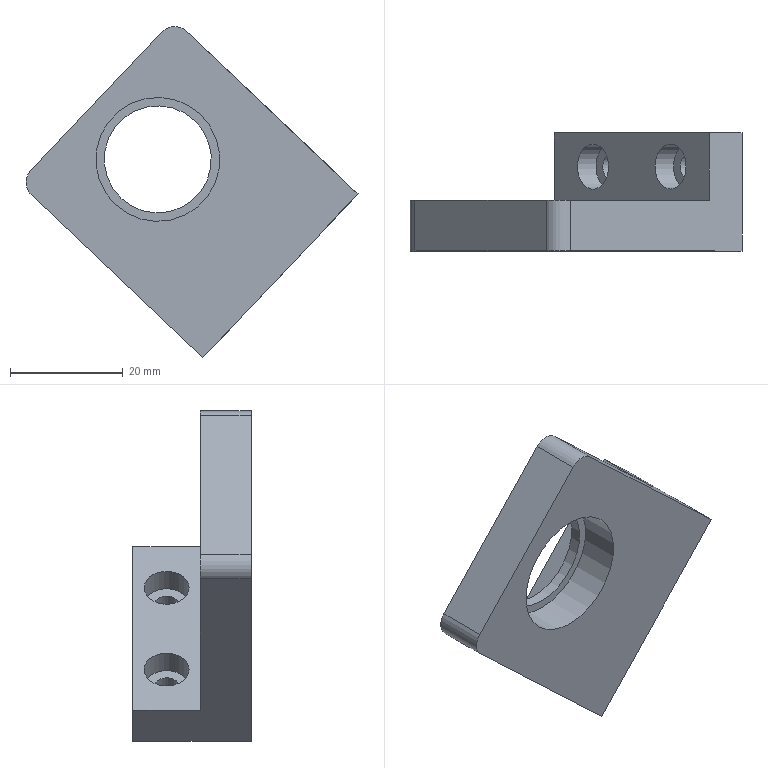Component | SolidWorks | 100-1_Copy(7)-1 | 1 solid | 25 faces | box 58.94 x 21 x 58.75 mm | volume 16214 mm3 | cylinder 14 | plane 11 | commonest cylinder face diameters 8 x4 4.5 x4 22 x2 6 x2 19 x2
STEP:
#1=COLOUR_RGB('',0.7922,0.8196,0.9333);
#2=FILL_AREA_STYLE_COLOUR('',#1);
#3=FILL_AREA_STYLE('',(#2));
#4=SURFACE_STYLE_FILL_AREA(#3);
#5=SURFACE_SIDE_STYLE('',(#4));
#6=SURFACE_STYLE_USAGE(.BOTH.,#5);
#7=PRESENTATION_STYLE_ASSIGNMENT((#6));
#8=CARTESIAN_POINT('',(19.833,50.,-78.793));
#9=VERTEX_POINT('',#8);
#10=CARTESIAN_POINT('',(19.319,50.,-79.336));
#11=VERTEX_POINT('',#10);
#12=CARTESIAN_POINT('',(19.576,50.,-79.065));
#13=DIRECTION('',(0.,-1.,-0.));
#14=DIRECTION('',(0.6879,0.,0.7258));
#15=AXIS2_PLACEMENT_3D('',#12,#13,#14);
#16=CIRCLE('',#15,0.374);
#17=EDGE_CURVE('',#9,#11,#16,.T.);
#18=ORIENTED_EDGE('',*,*,#17,.F.);
#19=CARTESIAN_POINT('',(19.576,50.,-79.065));
#20=DIRECTION('',(0.,-1.,-0.));
#21=DIRECTION('',(0.6879,0.,0.7258));
#22=AXIS2_PLACEMENT_3D('',#19,#20,#21);
#23=CIRCLE('',#22,0.374);
#24=EDGE_CURVE('',#11,#9,#23,.T.);
#25=ORIENTED_EDGE('',*,*,#24,.F.);
#26=EDGE_LOOP('',(#18,#25));
#27=FACE_BOUND('',#26,.T.);
#28=CARTESIAN_POINT('',(19.874,50.,-78.751));
#29=VERTEX_POINT('',#28);
#30=CARTESIAN_POINT('',(19.278,50.,-79.379));
#31=VERTEX_POINT('',#30);
#32=CARTESIAN_POINT('',(19.576,50.,-79.065));
#33=DIRECTION('',(0.,-1.,-0.));
#34=DIRECTION('',(0.6879,0.,0.7258));
#35=AXIS2_PLACEMENT_3D('',#32,#33,#34);
#36=CIRCLE('',#35,0.4331);
#37=EDGE_CURVE('',#29,#31,#36,.T.);
#38=ORIENTED_EDGE('',*,*,#37,.T.);
#39=CARTESIAN_POINT('',(19.576,50.,-79.065));
#40=DIRECTION('',(0.,-1.,-0.));
#41=DIRECTION('',(0.6879,0.,0.7258));
#42=AXIS2_PLACEMENT_3D('',#39,#40,#41);
#43=CIRCLE('',#42,0.4331);
#44=EDGE_CURVE('',#31,#29,#43,.T.);
#45=ORIENTED_EDGE('',*,*,#44,.T.);
#46=EDGE_LOOP('',(#38,#45));
#47=FACE_OUTER_BOUND('',#46,.T.);
#48=CARTESIAN_POINT('',(19.576,50.,-79.065));
#49=DIRECTION('',(0.,-1.,-0.));
#50=DIRECTION('',(0.7258,0.,-0.6879));
#51=AXIS2_PLACEMENT_3D('',#48,#49,#50);
#52=PLANE('',#51);
#53=ADVANCED_FACE('',(#27,#47),#52,.T.);
#54=CARTESIAN_POINT('',(19.278,49.724,-79.379));
#55=VERTEX_POINT('',#54);
#56=CARTESIAN_POINT('',(19.278,50.,-79.379));
#57=DIRECTION('',(0.,-1.,-0.));
#58=VECTOR('',#57,39.37);
#59=LINE('',#56,#58);
#60=EDGE_CURVE('',#31,#55,#59,.T.);
#61=ORIENTED_EDGE('',*,*,#60,.F.);
#62=ORIENTED_EDGE('',*,*,#37,.F.);
#63=CARTESIAN_POINT('',(19.874,49.724,-78.751));
#64=VERTEX_POINT('',#63);
#65=CARTESIAN_POINT('',(19.874,50.,-78.751));
#66=DIRECTION('',(0.,-1.,-0.));
#67=VECTOR('',#66,39.37);
#68=LINE('',#65,#67);
#69=EDGE_CURVE('',#29,#64,#68,.T.);
#70=ORIENTED_EDGE('',*,*,#69,.T.);
#71=CARTESIAN_POINT('',(19.576,49.724,-79.065));
#72=DIRECTION('',(0.,-1.,-0.));
#73=DIRECTION('',(0.6879,0.,0.7258));
#74=AXIS2_PLACEMENT_3D('',#71,#72,#73);
#75=CIRCLE('',#74,0.4331);
#76=EDGE_CURVE('',#64,#55,#75,.T.);
#77=ORIENTED_EDGE('',*,*,#76,.T.);
#78=EDGE_LOOP('',(#61,#62,#70,#77));
#79=FACE_OUTER_BOUND('',#78,.T.);
#80=CARTESIAN_POINT('',(19.576,50.,-79.065));
#81=DIRECTION('',(0.,-1.,-0.));
#82=DIRECTION('',(0.6879,0.,0.7258));
#83=AXIS2_PLACEMENT_3D('',#80,#81,#82);
#84=CYLINDRICAL_SURFACE('',#83,0.4331);
#85=ADVANCED_FACE('',(#79),#84,.F.);
#86=CARTESIAN_POINT('',(19.608,50.079,-78.173));
#87=VERTEX_POINT('',#86);
#88=CARTESIAN_POINT('',(19.775,50.079,-78.168));
#89=VERTEX_POINT('',#88);
#90=CARTESIAN_POINT('',(19.694,50.079,-78.254));
#91=DIRECTION('',(-0.,1.,0.));
#92=DIRECTION('',(-0.7258,0.,0.6879));
#93=AXIS2_PLACEMENT_3D('',#90,#91,#92);
#94=CIRCLE('',#93,0.1181);
#95=EDGE_CURVE('',#87,#89,#94,.T.);
#96=ORIENTED_EDGE('',*,*,#95,.F.);
#97=CARTESIAN_POINT('',(19.608,49.724,-78.173));
#98=VERTEX_POINT('',#97);
#99=CARTESIAN_POINT('',(19.608,50.551,-78.173));
#100=DIRECTION('',(-0.,1.,0.));
#101=VECTOR('',#100,39.37);
#102=LINE('',#99,#101);
#103=EDGE_CURVE('',#98,#87,#102,.T.);
#104=ORIENTED_EDGE('',*,*,#103,.F.);
#105=CARTESIAN_POINT('',(19.775,49.724,-78.168));
#106=VERTEX_POINT('',#105);
#107=CARTESIAN_POINT('',(19.694,49.724,-78.254));
#108=DIRECTION('',(0.,-1.,-0.));
#109=DIRECTION('',(0.6879,0.,0.7258));
#110=AXIS2_PLACEMENT_3D('',#107,#108,#109);
#111=CIRCLE('',#110,0.1181);
#112=EDGE_CURVE('',#106,#98,#111,.T.);
#113=ORIENTED_EDGE('',*,*,#112,.F.);
#114=CARTESIAN_POINT('',(19.775,50.551,-78.168));
#115=DIRECTION('',(0.,-1.,-0.));
#116=VECTOR('',#115,39.37);
#117=LINE('',#114,#116);
#118=EDGE_CURVE('',#89,#106,#117,.T.);
#119=ORIENTED_EDGE('',*,*,#118,.F.);
#120=EDGE_LOOP('',(#96,#104,#113,#119));
#121=FACE_OUTER_BOUND('',#120,.T.);
#122=CARTESIAN_POINT('',(19.694,50.551,-78.254));
#123=DIRECTION('',(0.,-1.,-0.));
#124=DIRECTION('',(0.6879,0.,0.7258));
#125=AXIS2_PLACEMENT_3D('',#122,#123,#124);
#126=CYLINDRICAL_SURFACE('',#125,0.1181);
#127=ADVANCED_FACE('',(#121),#126,.T.);
#128=CARTESIAN_POINT('',(18.692,50.079,-79.311));
#129=VERTEX_POINT('',#128);
#130=CARTESIAN_POINT('',(18.687,50.079,-79.145));
#131=VERTEX_POINT('',#130);
#132=CARTESIAN_POINT('',(18.773,50.079,-79.226));
#133=DIRECTION('',(-0.,1.,0.));
#134=DIRECTION('',(-0.7258,0.,0.6879));
#135=AXIS2_PLACEMENT_3D('',#132,#133,#134);
#136=CIRCLE('',#135,0.1181);
#137=EDGE_CURVE('',#129,#131,#136,.T.);
#138=ORIENTED_EDGE('',*,*,#137,.F.);
#139=CARTESIAN_POINT('',(18.692,49.724,-79.311));
#140=VERTEX_POINT('',#139);
#141=CARTESIAN_POINT('',(18.692,50.551,-79.311));
#142=DIRECTION('',(-0.,1.,0.));
#143=VECTOR('',#142,39.37);
#144=LINE('',#141,#143);
#145=EDGE_CURVE('',#140,#129,#144,.T.);
#146=ORIENTED_EDGE('',*,*,#145,.F.);
#147=CARTESIAN_POINT('',(18.687,49.724,-79.145));
#148=VERTEX_POINT('',#147);
#149=CARTESIAN_POINT('',(18.773,49.724,-79.226));
#150=DIRECTION('',(0.,-1.,-0.));
#151=DIRECTION('',(0.6879,0.,0.7258));
#152=AXIS2_PLACEMENT_3D('',#149,#150,#151);
#153=CIRCLE('',#152,0.1181);
#154=EDGE_CURVE('',#148,#140,#153,.T.);
#155=ORIENTED_EDGE('',*,*,#154,.F.);
#156=CARTESIAN_POINT('',(18.687,50.551,-79.145));
#157=DIRECTION('',(0.,-1.,-0.));
#158=VECTOR('',#157,39.37);
#159=LINE('',#156,#158);
#160=EDGE_CURVE('',#131,#148,#159,.T.);
#161=ORIENTED_EDGE('',*,*,#160,.F.);
#162=EDGE_LOOP('',(#138,#146,#155,#161));
#163=FACE_OUTER_BOUND('',#162,.T.);
#164=CARTESIAN_POINT('',(18.773,50.551,-79.226));
#165=DIRECTION('',(0.,-1.,-0.));
#166=DIRECTION('',(0.6879,0.,0.7258));
#167=AXIS2_PLACEMENT_3D('',#164,#165,#166);
#168=CYLINDRICAL_SURFACE('',#167,0.1181);
#169=ADVANCED_FACE('',(#163),#168,.T.);
#170=CARTESIAN_POINT('',(20.604,50.157,-79.497));
#171=VERTEX_POINT('',#170);
#172=CARTESIAN_POINT('',(20.476,50.157,-79.375));
#173=VERTEX_POINT('',#172);
#174=CARTESIAN_POINT('',(20.476,50.157,-79.375));
#175=DIRECTION('',(-0.7258,-0.,0.6879));
#176=VECTOR('',#175,39.37);
#177=LINE('',#174,#176);
#178=EDGE_CURVE('',#171,#173,#177,.T.);
#179=ORIENTED_EDGE('',*,*,#178,.F.);
#180=CARTESIAN_POINT('',(20.604,50.472,-79.497));
#181=VERTEX_POINT('',#180);
#182=CARTESIAN_POINT('',(20.604,50.315,-79.497));
#183=DIRECTION('',(-0.7258,-0.,0.6879));
#184=DIRECTION('',(0.,1.,0.));
#185=AXIS2_PLACEMENT_3D('',#182,#183,#184);
#186=CIRCLE('',#185,0.1575);
#187=EDGE_CURVE('',#181,#171,#186,.T.);
#188=ORIENTED_EDGE('',*,*,#187,.F.);
#189=CARTESIAN_POINT('',(20.476,50.472,-79.375));
#190=VERTEX_POINT('',#189);
#191=CARTESIAN_POINT('',(20.476,50.472,-79.375));
#192=DIRECTION('',(-0.7258,-0.,0.6879));
#193=VECTOR('',#192,39.37);
#194=LINE('',#191,#193);
#195=EDGE_CURVE('',#181,#190,#194,.T.);
#196=ORIENTED_EDGE('',*,*,#195,.T.);
#197=CARTESIAN_POINT('',(20.476,50.315,-79.375));
#198=DIRECTION('',(-0.7258,-0.,0.6879));
#199=DIRECTION('',(0.,1.,0.));
#200=AXIS2_PLACEMENT_3D('',#197,#198,#199);
#201=CIRCLE('',#200,0.1575);
#202=EDGE_CURVE('',#190,#173,#201,.T.);
#203=ORIENTED_EDGE('',*,*,#202,.T.);
#204=EDGE_LOOP('',(#179,#188,#196,#203));
#205=FACE_OUTER_BOUND('',#204,.T.);
#206=CARTESIAN_POINT('',(20.476,50.315,-79.375));
#207=DIRECTION('',(-0.7258,-0.,0.6879));
#208=DIRECTION('',(0.,1.,0.));
#209=AXIS2_PLACEMENT_3D('',#206,#207,#208);
#210=CYLINDRICAL_SURFACE('',#209,0.1575);
#211=ADVANCED_FACE('',(#205),#210,.F.);
#212=CARTESIAN_POINT('',(20.604,50.404,-79.497));
#213=VERTEX_POINT('',#212);
#214=CARTESIAN_POINT('',(20.604,50.226,-79.497));
#215=VERTEX_POINT('',#214);
#216=CARTESIAN_POINT('',(20.604,50.315,-79.497));
#217=DIRECTION('',(-0.7258,-0.,0.6879));
#218=DIRECTION('',(0.,1.,0.));
#219=AXIS2_PLACEMENT_3D('',#216,#217,#218);
#220=CIRCLE('',#219,0.08858);
#221=EDGE_CURVE('',#213,#215,#220,.T.);
#222=ORIENTED_EDGE('',*,*,#221,.F.);
#223=CARTESIAN_POINT('',(20.604,50.315,-79.497));
#224=DIRECTION('',(-0.7258,-0.,0.6879));
#225=DIRECTION('',(0.,1.,0.));
#226=AXIS2_PLACEMENT_3D('',#223,#224,#225);
#227=CIRCLE('',#226,0.08858);
#228=EDGE_CURVE('',#215,#213,#227,.T.);
#229=ORIENTED_EDGE('',*,*,#228,.F.);
#230=EDGE_LOOP('',(#222,#229));
#231=FACE_BOUND('',#230,.T.);
#232=ORIENTED_EDGE('',*,*,#187,.T.);
#233=CARTESIAN_POINT('',(20.604,50.315,-79.497));
#234=DIRECTION('',(-0.7258,-0.,0.6879));
#235=DIRECTION('',(0.,1.,0.));
#236=AXIS2_PLACEMENT_3D('',#233,#234,#235);
#237=CIRCLE('',#236,0.1575);
#238=EDGE_CURVE('',#171,#181,#237,.T.);
#239=ORIENTED_EDGE('',*,*,#238,.T.);
#240=EDGE_LOOP('',(#232,#239));
#241=FACE_OUTER_BOUND('',#240,.T.);
#242=CARTESIAN_POINT('',(20.543,50.315,-79.561));
#243=DIRECTION('',(0.7258,0.,-0.6879));
#244=DIRECTION('',(0.6879,0.,0.7258));
#245=AXIS2_PLACEMENT_3D('',#242,#243,#244);
#246=PLANE('',#245);
#247=ADVANCED_FACE('',(#231,#241),#246,.F.);
#248=CARTESIAN_POINT('',(20.704,50.226,-79.592));
#249=VERTEX_POINT('',#248);
#250=CARTESIAN_POINT('',(20.476,50.226,-79.375));
#251=DIRECTION('',(-0.7258,-0.,0.6879));
#252=VECTOR('',#251,39.37);
#253=LINE('',#250,#252);
#254=EDGE_CURVE('',#249,#215,#253,.T.);
#255=ORIENTED_EDGE('',*,*,#254,.F.);
#256=CARTESIAN_POINT('',(20.704,50.404,-79.592));
#257=VERTEX_POINT('',#256);
#258=CARTESIAN_POINT('',(20.704,50.315,-79.592));
#259=DIRECTION('',(-0.7258,-0.,0.6879));
#260=DIRECTION('',(0.,1.,0.));
#261=AXIS2_PLACEMENT_3D('',#258,#259,#260);
#262=CIRCLE('',#261,0.08858);
#263=EDGE_CURVE('',#257,#249,#262,.T.);
#264=ORIENTED_EDGE('',*,*,#263,.F.);
#265=CARTESIAN_POINT('',(20.476,50.404,-79.375));
#266=DIRECTION('',(-0.7258,-0.,0.6879));
#267=VECTOR('',#266,39.37);
#268=LINE('',#265,#267);
#269=EDGE_CURVE('',#257,#213,#268,.T.);
#270=ORIENTED_EDGE('',*,*,#269,.T.);
#271=ORIENTED_EDGE('',*,*,#221,.T.);
#272=EDGE_LOOP('',(#255,#264,#270,#271));
#273=FACE_OUTER_BOUND('',#272,.T.);
#274=CARTESIAN_POINT('',(20.476,50.315,-79.375));
#275=DIRECTION('',(-0.7258,-0.,0.6879));
#276=DIRECTION('',(0.,1.,0.));
#277=AXIS2_PLACEMENT_3D('',#274,#275,#276);
#278=CYLINDRICAL_SURFACE('',#277,0.08858);
#279=ADVANCED_FACE('',(#273),#278,.F.);
#280=CARTESIAN_POINT('',(20.063,50.157,-80.068));
#281=VERTEX_POINT('',#280);
#282=CARTESIAN_POINT('',(19.934,50.157,-79.946));
#283=VERTEX_POINT('',#282);
#284=CARTESIAN_POINT('',(19.934,50.157,-79.946));
#285=DIRECTION('',(-0.7258,-0.,0.6879));
#286=VECTOR('',#285,39.37);
#287=LINE('',#284,#286);
#288=EDGE_CURVE('',#281,#283,#287,.T.);
#289=ORIENTED_EDGE('',*,*,#288,.F.);
#290=CARTESIAN_POINT('',(20.063,50.472,-80.068));
#291=VERTEX_POINT('',#290);
#292=CARTESIAN_POINT('',(20.063,50.315,-80.068));
#293=DIRECTION('',(-0.7258,-0.,0.6879));
#294=DIRECTION('',(0.,1.,0.));
#295=AXIS2_PLACEMENT_3D('',#292,#293,#294);
#296=CIRCLE('',#295,0.1575);
#297=EDGE_CURVE('',#291,#281,#296,.T.);
#298=ORIENTED_EDGE('',*,*,#297,.F.);
#299=CARTESIAN_POINT('',(19.934,50.472,-79.946));
#300=VERTEX_POINT('',#299);
#301=CARTESIAN_POINT('',(19.934,50.472,-79.946));
#302=DIRECTION('',(-0.7258,-0.,0.6879));
#303=VECTOR('',#302,39.37);
#304=LINE('',#301,#303);
#305=EDGE_CURVE('',#291,#300,#304,.T.);
#306=ORIENTED_EDGE('',*,*,#305,.T.);
#307=CARTESIAN_POINT('',(19.934,50.315,-79.946));
#308=DIRECTION('',(-0.7258,-0.,0.6879));
#309=DIRECTION('',(0.,1.,0.));
#310=AXIS2_PLACEMENT_3D('',#307,#308,#309);
#311=CIRCLE('',#310,0.1575);
#312=EDGE_CURVE('',#300,#283,#311,.T.);
#313=ORIENTED_EDGE('',*,*,#312,.T.);
#314=EDGE_LOOP('',(#289,#298,#306,#313));
#315=FACE_OUTER_BOUND('',#314,.T.);
#316=CARTESIAN_POINT('',(19.934,50.315,-79.946));
#317=DIRECTION('',(-0.7258,-0.,0.6879));
#318=DIRECTION('',(0.,1.,0.));
#319=AXIS2_PLACEMENT_3D('',#316,#317,#318);
#320=CYLINDRICAL_SURFACE('',#319,0.1575);
#321=ADVANCED_FACE('',(#315),#320,.F.);
#322=CARTESIAN_POINT('',(20.063,50.404,-80.068));
#323=VERTEX_POINT('',#322);
#324=CARTESIAN_POINT('',(20.063,50.226,-80.068));
#325=VERTEX_POINT('',#324);
#326=CARTESIAN_POINT('',(20.063,50.315,-80.068));
#327=DIRECTION('',(-0.7258,-0.,0.6879));
#328=DIRECTION('',(0.,1.,0.));
#329=AXIS2_PLACEMENT_3D('',#326,#327,#328);
#330=CIRCLE('',#329,0.08858);
#331=EDGE_CURVE('',#323,#325,#330,.T.);
#332=ORIENTED_EDGE('',*,*,#331,.F.);
#333=CARTESIAN_POINT('',(20.063,50.315,-80.068));
#334=DIRECTION('',(-0.7258,-0.,0.6879));
#335=DIRECTION('',(0.,1.,0.));
#336=AXIS2_PLACEMENT_3D('',#333,#334,#335);
#337=CIRCLE('',#336,0.08858);
#338=EDGE_CURVE('',#325,#323,#337,.T.);
#339=ORIENTED_EDGE('',*,*,#338,.F.);
#340=EDGE_LOOP('',(#332,#339));
#341=FACE_BOUND('',#340,.T.);
#342=ORIENTED_EDGE('',*,*,#297,.T.);
#343=CARTESIAN_POINT('',(20.063,50.315,-80.068));
#344=DIRECTION('',(-0.7258,-0.,0.6879));
#345=DIRECTION('',(0.,1.,0.));
#346=AXIS2_PLACEMENT_3D('',#343,#344,#345);
#347=CIRCLE('',#346,0.1575);
#348=EDGE_CURVE('',#281,#291,#347,.T.);
#349=ORIENTED_EDGE('',*,*,#348,.T.);
#350=EDGE_LOOP('',(#342,#349));
#351=FACE_OUTER_BOUND('',#350,.T.);
#352=CARTESIAN_POINT('',(20.002,50.315,-80.133));
#353=DIRECTION('',(0.7258,0.,-0.6879));
#354=DIRECTION('',(0.6879,0.,0.7258));
#355=AXIS2_PLACEMENT_3D('',#352,#353,#354);
#356=PLANE('',#355);
#357=ADVANCED_FACE('',(#341,#351),#356,.F.);
#358=CARTESIAN_POINT('',(20.163,50.226,-80.163));
#359=VERTEX_POINT('',#358);
#360=CARTESIAN_POINT('',(19.934,50.226,-79.946));
#361=DIRECTION('',(-0.7258,-0.,0.6879));
#362=VECTOR('',#361,39.37);
#363=LINE('',#360,#362);
#364=EDGE_CURVE('',#359,#325,#363,.T.);
#365=ORIENTED_EDGE('',*,*,#364,.F.);
#366=CARTESIAN_POINT('',(20.163,50.404,-80.163));
#367=VERTEX_POINT('',#366);
#368=CARTESIAN_POINT('',(20.163,50.315,-80.163));
#369=DIRECTION('',(-0.7258,-0.,0.6879));
#370=DIRECTION('',(0.,1.,0.));
#371=AXIS2_PLACEMENT_3D('',#368,#369,#370);
#372=CIRCLE('',#371,0.08858);
#373=EDGE_CURVE('',#367,#359,#372,.T.);
#374=ORIENTED_EDGE('',*,*,#373,.F.);
#375=CARTESIAN_POINT('',(19.934,50.404,-79.946));
#376=DIRECTION('',(-0.7258,-0.,0.6879));
#377=VECTOR('',#376,39.37);
#378=LINE('',#375,#377);
#379=EDGE_CURVE('',#367,#323,#378,.T.);
#380=ORIENTED_EDGE('',*,*,#379,.T.);
#381=ORIENTED_EDGE('',*,*,#331,.T.);
#382=EDGE_LOOP('',(#365,#374,#380,#381));
#383=FACE_OUTER_BOUND('',#382,.T.);
#384=CARTESIAN_POINT('',(19.934,50.315,-79.946));
#385=DIRECTION('',(-0.7258,-0.,0.6879));
#386=DIRECTION('',(0.,1.,0.));
#387=AXIS2_PLACEMENT_3D('',#384,#385,#386);
#388=CYLINDRICAL_SURFACE('',#387,0.08858);
#389=ADVANCED_FACE('',(#383),#388,.F.);
#390=ORIENTED_EDGE('',*,*,#312,.F.);
#391=CARTESIAN_POINT('',(19.934,50.315,-79.946));
#392=DIRECTION('',(-0.7258,-0.,0.6879));
#393=DIRECTION('',(0.,1.,0.));
#394=AXIS2_PLACEMENT_3D('',#391,#392,#393);
#395=CIRCLE('',#394,0.1575);
#396=EDGE_CURVE('',#283,#300,#395,.T.);
#397=ORIENTED_EDGE('',*,*,#396,.F.);
#398=EDGE_LOOP('',(#390,#397));
#399=FACE_BOUND('',#398,.T.);
#400=ORIENTED_EDGE('',*,*,#202,.F.);
#401=CARTESIAN_POINT('',(20.476,50.315,-79.375));
#402=DIRECTION('',(-0.7258,-0.,0.6879));
#403=DIRECTION('',(0.,1.,0.));
#404=AXIS2_PLACEMENT_3D('',#401,#402,#403);
#405=CIRCLE('',#404,0.1575);
#406=EDGE_CURVE('',#173,#190,#405,.T.);
#407=ORIENTED_EDGE('',*,*,#406,.F.);
#408=EDGE_LOOP('',(#400,#407));
#409=FACE_BOUND('',#408,.T.);
#410=CARTESIAN_POINT('',(19.663,50.551,-80.232));
#411=VERTEX_POINT('',#410);
#412=CARTESIAN_POINT('',(19.663,50.079,-80.232));
#413=VERTEX_POINT('',#412);
#414=CARTESIAN_POINT('',(19.663,50.551,-80.232));
#415=DIRECTION('',(0.,-1.,-0.));
#416=VECTOR('',#415,39.37);
#417=LINE('',#414,#416);
#418=EDGE_CURVE('',#411,#413,#417,.T.);
#419=ORIENTED_EDGE('',*,*,#418,.T.);
#420=CARTESIAN_POINT('',(20.746,50.079,-79.089));
#421=VERTEX_POINT('',#420);
#422=CARTESIAN_POINT('',(20.746,50.079,-79.089));
#423=DIRECTION('',(-0.6879,-0.,-0.7258));
#424=VECTOR('',#423,39.37);
#425=LINE('',#422,#424);
#426=EDGE_CURVE('',#421,#413,#425,.T.);
#427=ORIENTED_EDGE('',*,*,#426,.F.);
#428=CARTESIAN_POINT('',(20.746,50.551,-79.089));
#429=VERTEX_POINT('',#428);
#430=CARTESIAN_POINT('',(20.746,50.551,-79.089));
#431=DIRECTION('',(0.,-1.,-0.));
#432=VECTOR('',#431,39.37);
#433=LINE('',#430,#432);
#434=EDGE_CURVE('',#429,#421,#433,.T.);
#435=ORIENTED_EDGE('',*,*,#434,.F.);
#436=CARTESIAN_POINT('',(20.746,50.551,-79.089));
#437=DIRECTION('',(-0.6879,-0.,-0.7258));
#438=VECTOR('',#437,39.37);
#439=LINE('',#436,#438);
#440=EDGE_CURVE('',#429,#411,#439,.T.);
#441=ORIENTED_EDGE('',*,*,#440,.T.);
#442=EDGE_LOOP('',(#419,#427,#435,#441));
#443=FACE_OUTER_BOUND('',#442,.T.);
#444=CARTESIAN_POINT('',(20.746,50.551,-79.089));
#445=DIRECTION('',(0.7258,0.,-0.6879));
#446=DIRECTION('',(0.,-1.,-0.));
#447=AXIS2_PLACEMENT_3D('',#444,#445,#446);
#448=PLANE('',#447);
#449=ADVANCED_FACE('',(#399,#409,#443),#448,.F.);
#450=CARTESIAN_POINT('',(19.833,50.079,-78.793));
#451=VERTEX_POINT('',#450);
#452=CARTESIAN_POINT('',(19.319,50.079,-79.336));
#453=VERTEX_POINT('',#452);
#454=CARTESIAN_POINT('',(19.576,50.079,-79.065));
#455=DIRECTION('',(0.,-1.,-0.));
#456=DIRECTION('',(-0.7258,0.,0.6879));
#457=AXIS2_PLACEMENT_3D('',#454,#455,#456);
#458=CIRCLE('',#457,0.374);
#459=EDGE_CURVE('',#451,#453,#458,.T.);
#460=ORIENTED_EDGE('',*,*,#459,.T.);
#461=CARTESIAN_POINT('',(19.576,50.079,-79.065));
#462=DIRECTION('',(0.,-1.,-0.));
#463=DIRECTION('',(-0.7258,0.,0.6879));
#464=AXIS2_PLACEMENT_3D('',#461,#462,#463);
#465=CIRCLE('',#464,0.374);
#466=EDGE_CURVE('',#453,#451,#465,.T.);
#467=ORIENTED_EDGE('',*,*,#466,.T.);
#468=EDGE_LOOP('',(#460,#467));
#469=FACE_BOUND('',#468,.T.);
#470=CARTESIAN_POINT('',(18.606,50.079,-79.23));
#471=DIRECTION('',(-0.7258,-0.,0.6879));
#472=VECTOR('',#471,39.37);
#473=LINE('',#470,#472);
#474=EDGE_CURVE('',#413,#129,#473,.T.);
#475=ORIENTED_EDGE('',*,*,#474,.T.);
#476=ORIENTED_EDGE('',*,*,#137,.T.);
#477=CARTESIAN_POINT('',(19.689,50.079,-78.087));
#478=DIRECTION('',(-0.6879,-0.,-0.7258));
#479=VECTOR('',#478,39.37);
#480=LINE('',#477,#479);
#481=EDGE_CURVE('',#87,#131,#480,.T.);
#482=ORIENTED_EDGE('',*,*,#481,.F.);
#483=ORIENTED_EDGE('',*,*,#95,.T.);
#484=CARTESIAN_POINT('',(19.689,50.079,-78.087));
#485=DIRECTION('',(-0.7258,-0.,0.6879));
#486=VECTOR('',#485,39.37);
#487=LINE('',#484,#486);
#488=EDGE_CURVE('',#421,#89,#487,.T.);
#489=ORIENTED_EDGE('',*,*,#488,.F.);
#490=ORIENTED_EDGE('',*,*,#426,.T.);
#491=EDGE_LOOP('',(#475,#476,#482,#483,#489,#490));
#492=FACE_OUTER_BOUND('',#491,.T.);
#493=CARTESIAN_POINT('',(19.689,50.079,-78.087));
#494=DIRECTION('',(0.,-1.,-0.));
#495=DIRECTION('',(0.6879,0.,0.7258));
#496=AXIS2_PLACEMENT_3D('',#493,#494,#495);
#497=PLANE('',#496);
#498=ADVANCED_FACE('',(#469,#492),#497,.F.);
#499=ORIENTED_EDGE('',*,*,#373,.T.);
#500=CARTESIAN_POINT('',(20.163,50.315,-80.163));
#501=DIRECTION('',(-0.7258,-0.,0.6879));
#502=DIRECTION('',(0.,1.,0.));
#503=AXIS2_PLACEMENT_3D('',#500,#501,#502);
#504=CIRCLE('',#503,0.08858);
#505=EDGE_CURVE('',#359,#367,#504,.T.);
#506=ORIENTED_EDGE('',*,*,#505,.T.);
#507=EDGE_LOOP('',(#499,#506));
#508=FACE_BOUND('',#507,.T.);
#509=ORIENTED_EDGE('',*,*,#263,.T.);
#510=CARTESIAN_POINT('',(20.704,50.315,-79.592));
#511=DIRECTION('',(-0.7258,-0.,0.6879));
#512=DIRECTION('',(0.,1.,0.));
#513=AXIS2_PLACEMENT_3D('',#510,#511,#512);
#514=CIRCLE('',#513,0.08858);
#515=EDGE_CURVE('',#249,#257,#514,.T.);
#516=ORIENTED_EDGE('',*,*,#515,.T.);
#517=EDGE_LOOP('',(#509,#516));
#518=FACE_BOUND('',#517,.T.);
#519=CARTESIAN_POINT('',(20.975,49.724,-79.306));
#520=VERTEX_POINT('',#519);
#521=CARTESIAN_POINT('',(19.892,49.724,-80.449));
#522=VERTEX_POINT('',#521);
#523=CARTESIAN_POINT('',(20.975,49.724,-79.306));
#524=DIRECTION('',(-0.6879,-0.,-0.7258));
#525=VECTOR('',#524,39.37);
#526=LINE('',#523,#525);
#527=EDGE_CURVE('',#520,#522,#526,.T.);
#528=ORIENTED_EDGE('',*,*,#527,.T.);
#529=CARTESIAN_POINT('',(19.892,50.551,-80.449));
#530=VERTEX_POINT('',#529);
#531=CARTESIAN_POINT('',(19.892,50.551,-80.449));
#532=DIRECTION('',(0.,-1.,-0.));
#533=VECTOR('',#532,39.37);
#534=LINE('',#531,#533);
#535=EDGE_CURVE('',#530,#522,#534,.T.);
#536=ORIENTED_EDGE('',*,*,#535,.F.);
#537=CARTESIAN_POINT('',(20.975,50.551,-79.306));
#538=VERTEX_POINT('',#537);
#539=CARTESIAN_POINT('',(20.975,50.551,-79.306));
#540=DIRECTION('',(-0.6879,-0.,-0.7258));
#541=VECTOR('',#540,39.37);
#542=LINE('',#539,#541);
#543=EDGE_CURVE('',#538,#530,#542,.T.);
#544=ORIENTED_EDGE('',*,*,#543,.F.);
#545=CARTESIAN_POINT('',(20.975,50.551,-79.306));
#546=DIRECTION('',(0.,-1.,-0.));
#547=VECTOR('',#546,39.37);
#548=LINE('',#545,#547);
#549=EDGE_CURVE('',#538,#520,#548,.T.);
#550=ORIENTED_EDGE('',*,*,#549,.T.);
#551=EDGE_LOOP('',(#528,#536,#544,#550));
#552=FACE_OUTER_BOUND('',#551,.T.);
#553=CARTESIAN_POINT('',(20.975,50.551,-79.306));
#554=DIRECTION('',(-0.7258,-0.,0.6879));
#555=DIRECTION('',(-0.6879,-0.,-0.7258));
#556=AXIS2_PLACEMENT_3D('',#553,#554,#555);
#557=PLANE('',#556);
#558=ADVANCED_FACE('',(#508,#518,#552),#557,.F.);
#559=ORIENTED_EDGE('',*,*,#488,.T.);
#560=ORIENTED_EDGE('',*,*,#118,.T.);
#561=CARTESIAN_POINT('',(20.975,49.724,-79.306));
#562=DIRECTION('',(0.7258,0.,-0.6879));
#563=VECTOR('',#562,39.37);
#564=LINE('',#561,#563);
#565=EDGE_CURVE('',#106,#520,#564,.T.);
#566=ORIENTED_EDGE('',*,*,#565,.T.);
#567=ORIENTED_EDGE('',*,*,#549,.F.);
#568=CARTESIAN_POINT('',(20.975,50.551,-79.306));
#569=DIRECTION('',(0.7258,0.,-0.6879));
#570=VECTOR('',#569,39.37);
#571=LINE('',#568,#570);
#572=EDGE_CURVE('',#429,#538,#571,.T.);
#573=ORIENTED_EDGE('',*,*,#572,.F.);
#574=ORIENTED_EDGE('',*,*,#434,.T.);
#575=EDGE_LOOP('',(#559,#560,#566,#567,#573,#574));
#576=FACE_OUTER_BOUND('',#575,.T.);
#577=CARTESIAN_POINT('',(20.975,50.551,-79.306));
#578=DIRECTION('',(-0.6879,-0.,-0.7258));
#579=DIRECTION('',(-0.7258,-0.,0.6879));
#580=AXIS2_PLACEMENT_3D('',#577,#578,#579);
#581=PLANE('',#580);
#582=ADVANCED_FACE('',(#576),#581,.F.);
#583=ORIENTED_EDGE('',*,*,#481,.T.);
#584=ORIENTED_EDGE('',*,*,#160,.T.);
#585=CARTESIAN_POINT('',(19.689,49.724,-78.087));
#586=DIRECTION('',(0.6879,0.,0.7258));
#587=VECTOR('',#586,39.37);
#588=LINE('',#585,#587);
#589=EDGE_CURVE('',#148,#98,#588,.T.);
#590=ORIENTED_EDGE('',*,*,#589,.T.);
#591=ORIENTED_EDGE('',*,*,#103,.T.);
#592=EDGE_LOOP('',(#583,#584,#590,#591));
#593=FACE_OUTER_BOUND('',#592,.T.);
#594=CARTESIAN_POINT('',(19.689,50.551,-78.087));
#595=DIRECTION('',(0.7258,0.,-0.6879));
#596=DIRECTION('',(0.,-1.,-0.));
#597=AXIS2_PLACEMENT_3D('',#594,#595,#596);
#598=PLANE('',#597);
#599=ADVANCED_FACE('',(#593),#598,.F.);
#600=CARTESIAN_POINT('',(19.892,49.724,-80.449));
#601=DIRECTION('',(-0.7258,-0.,0.6879));
#602=VECTOR('',#601,39.37);
#603=LINE('',#600,#602);
#604=EDGE_CURVE('',#522,#140,#603,.T.);
#605=ORIENTED_EDGE('',*,*,#604,.T.);
#606=ORIENTED_EDGE('',*,*,#145,.T.);
#607=ORIENTED_EDGE('',*,*,#474,.F.);
#608=ORIENTED_EDGE('',*,*,#418,.F.);
#609=CARTESIAN_POINT('',(19.892,50.551,-80.449));
#610=DIRECTION('',(-0.7258,-0.,0.6879));
#611=VECTOR('',#610,39.37);
#612=LINE('',#609,#611);
#613=EDGE_CURVE('',#530,#411,#612,.T.);
#614=ORIENTED_EDGE('',*,*,#613,.F.);
#615=ORIENTED_EDGE('',*,*,#535,.T.);
#616=EDGE_LOOP('',(#605,#606,#607,#608,#614,#615));
#617=FACE_OUTER_BOUND('',#616,.T.);
#618=CARTESIAN_POINT('',(19.892,50.551,-80.449));
#619=DIRECTION('',(0.6879,0.,0.7258));
#620=DIRECTION('',(-0.,1.,0.));
#621=AXIS2_PLACEMENT_3D('',#618,#619,#620);
#622=PLANE('',#621);
#623=ADVANCED_FACE('',(#617),#622,.F.);
#624=ORIENTED_EDGE('',*,*,#76,.F.);
#625=CARTESIAN_POINT('',(19.576,49.724,-79.065));
#626=DIRECTION('',(0.,-1.,-0.));
#627=DIRECTION('',(0.6879,0.,0.7258));
#628=AXIS2_PLACEMENT_3D('',#625,#626,#627);
#629=CIRCLE('',#628,0.4331);
#630=EDGE_CURVE('',#55,#64,#629,.T.);
#631=ORIENTED_EDGE('',*,*,#630,.F.);
#632=EDGE_LOOP('',(#624,#631));
#633=FACE_BOUND('',#632,.T.);
#634=ORIENTED_EDGE('',*,*,#589,.F.);
#635=ORIENTED_EDGE('',*,*,#154,.T.);
#636=ORIENTED_EDGE('',*,*,#604,.F.);
#637=ORIENTED_EDGE('',*,*,#527,.F.);
#638=ORIENTED_EDGE('',*,*,#565,.F.);
#639=ORIENTED_EDGE('',*,*,#112,.T.);
#640=EDGE_LOOP('',(#634,#635,#636,#637,#638,#639));
#641=FACE_OUTER_BOUND('',#640,.T.);
#642=CARTESIAN_POINT('',(19.79,49.724,-79.268));
#643=DIRECTION('',(0.,-1.,-0.));
#644=DIRECTION('',(0.7258,0.,-0.6879));
#645=AXIS2_PLACEMENT_3D('',#642,#643,#644);
#646=PLANE('',#645);
#647=ADVANCED_FACE('',(#633,#641),#646,.T.);
#648=ORIENTED_EDGE('',*,*,#613,.T.);
#649=ORIENTED_EDGE('',*,*,#440,.F.);
#650=ORIENTED_EDGE('',*,*,#572,.T.);
#651=ORIENTED_EDGE('',*,*,#543,.T.);
#652=EDGE_LOOP('',(#648,#649,#650,#651));
#653=FACE_OUTER_BOUND('',#652,.T.);
#654=CARTESIAN_POINT('',(19.79,50.551,-79.268));
#655=DIRECTION('',(0.,-1.,-0.));
#656=DIRECTION('',(0.7258,0.,-0.6879));
#657=AXIS2_PLACEMENT_3D('',#654,#655,#656);
#658=PLANE('',#657);
#659=ADVANCED_FACE('',(#653),#658,.F.);
#660=CARTESIAN_POINT('',(19.319,50.551,-79.336));
#661=DIRECTION('',(0.,-1.,-0.));
#662=VECTOR('',#661,39.37);
#663=LINE('',#660,#662);
#664=EDGE_CURVE('',#453,#11,#663,.T.);
#665=ORIENTED_EDGE('',*,*,#664,.F.);
#666=ORIENTED_EDGE('',*,*,#459,.F.);
#667=CARTESIAN_POINT('',(19.833,50.551,-78.793));
#668=DIRECTION('',(0.,-1.,-0.));
#669=VECTOR('',#668,39.37);
#670=LINE('',#667,#669);
#671=EDGE_CURVE('',#451,#9,#670,.T.);
#672=ORIENTED_EDGE('',*,*,#671,.T.);
#673=ORIENTED_EDGE('',*,*,#17,.T.);
#674=EDGE_LOOP('',(#665,#666,#672,#673));
#675=FACE_OUTER_BOUND('',#674,.T.);
#676=CARTESIAN_POINT('',(19.576,50.551,-79.065));
#677=DIRECTION('',(0.,-1.,-0.));
#678=DIRECTION('',(0.6879,0.,0.7258));
#679=AXIS2_PLACEMENT_3D('',#676,#677,#678);
#680=CYLINDRICAL_SURFACE('',#679,0.374);
#681=ADVANCED_FACE('',(#675),#680,.F.);
#682=ORIENTED_EDGE('',*,*,#466,.F.);
#683=ORIENTED_EDGE('',*,*,#664,.T.);
#684=ORIENTED_EDGE('',*,*,#24,.T.);
#685=ORIENTED_EDGE('',*,*,#671,.F.);
#686=EDGE_LOOP('',(#682,#683,#684,#685));
#687=FACE_OUTER_BOUND('',#686,.T.);
#688=CARTESIAN_POINT('',(19.576,50.551,-79.065));
#689=DIRECTION('',(0.,-1.,-0.));
#690=DIRECTION('',(0.6879,0.,0.7258));
#691=AXIS2_PLACEMENT_3D('',#688,#689,#690);
#692=CYLINDRICAL_SURFACE('',#691,0.374);
#693=ADVANCED_FACE('',(#687),#692,.F.);
#694=ORIENTED_EDGE('',*,*,#505,.F.);
#695=ORIENTED_EDGE('',*,*,#364,.T.);
#696=ORIENTED_EDGE('',*,*,#338,.T.);
#697=ORIENTED_EDGE('',*,*,#379,.F.);
#698=EDGE_LOOP('',(#694,#695,#696,#697));
#699=FACE_OUTER_BOUND('',#698,.T.);
#700=CARTESIAN_POINT('',(19.934,50.315,-79.946));
#701=DIRECTION('',(-0.7258,-0.,0.6879));
#702=DIRECTION('',(0.,1.,0.));
#703=AXIS2_PLACEMENT_3D('',#700,#701,#702);
#704=CYLINDRICAL_SURFACE('',#703,0.08858);
#705=ADVANCED_FACE('',(#699),#704,.F.);
#706=ORIENTED_EDGE('',*,*,#348,.F.);
#707=ORIENTED_EDGE('',*,*,#288,.T.);
#708=ORIENTED_EDGE('',*,*,#396,.T.);
#709=ORIENTED_EDGE('',*,*,#305,.F.);
#710=EDGE_LOOP('',(#706,#707,#708,#709));
#711=FACE_OUTER_BOUND('',#710,.T.);
#712=CARTESIAN_POINT('',(19.934,50.315,-79.946));
#713=DIRECTION('',(-0.7258,-0.,0.6879));
#714=DIRECTION('',(0.,1.,0.));
#715=AXIS2_PLACEMENT_3D('',#712,#713,#714);
#716=CYLINDRICAL_SURFACE('',#715,0.1575);
#717=ADVANCED_FACE('',(#711),#716,.F.);
#718=ORIENTED_EDGE('',*,*,#515,.F.);
#719=ORIENTED_EDGE('',*,*,#254,.T.);
#720=ORIENTED_EDGE('',*,*,#228,.T.);
#721=ORIENTED_EDGE('',*,*,#269,.F.);
#722=EDGE_LOOP('',(#718,#719,#720,#721));
#723=FACE_OUTER_BOUND('',#722,.T.);
#724=CARTESIAN_POINT('',(20.476,50.315,-79.375));
#725=DIRECTION('',(-0.7258,-0.,0.6879));
#726=DIRECTION('',(0.,1.,0.));
#727=AXIS2_PLACEMENT_3D('',#724,#725,#726);
#728=CYLINDRICAL_SURFACE('',#727,0.08858);
#729=ADVANCED_FACE('',(#723),#728,.F.);
#730=ORIENTED_EDGE('',*,*,#238,.F.);
#731=ORIENTED_EDGE('',*,*,#178,.T.);
#732=ORIENTED_EDGE('',*,*,#406,.T.);
#733=ORIENTED_EDGE('',*,*,#195,.F.);
#734=EDGE_LOOP('',(#730,#731,#732,#733));
#735=FACE_OUTER_BOUND('',#734,.T.);
#736=CARTESIAN_POINT('',(20.476,50.315,-79.375));
#737=DIRECTION('',(-0.7258,-0.,0.6879));
#738=DIRECTION('',(0.,1.,0.));
#739=AXIS2_PLACEMENT_3D('',#736,#737,#738);
#740=CYLINDRICAL_SURFACE('',#739,0.1575);
#741=ADVANCED_FACE('',(#735),#740,.F.);
#742=ORIENTED_EDGE('',*,*,#44,.F.);
#743=ORIENTED_EDGE('',*,*,#60,.T.);
#744=ORIENTED_EDGE('',*,*,#630,.T.);
#745=ORIENTED_EDGE('',*,*,#69,.F.);
#746=EDGE_LOOP('',(#742,#743,#744,#745));
#747=FACE_OUTER_BOUND('',#746,.T.);
#748=CARTESIAN_POINT('',(19.576,50.,-79.065));
#749=DIRECTION('',(0.,-1.,-0.));
#750=DIRECTION('',(0.6879,0.,0.7258));
#751=AXIS2_PLACEMENT_3D('',#748,#749,#750);
#752=CYLINDRICAL_SURFACE('',#751,0.4331);
#753=ADVANCED_FACE('',(#747),#752,.F.);
#754=CLOSED_SHELL('',(#53,#85,#127,#169,#211,#247,#279,#321,#357,#389,#449,#498,#558,#582,#599,#623,#647,#659,#681,#693,#705,#717,#729,#741,#753));
#755=MANIFOLD_SOLID_BREP('',#754);
#756=STYLED_ITEM('',(#7),#755);
#757=(LENGTH_UNIT()NAMED_UNIT(*)SI_UNIT($,.METRE.));
#758=LENGTH_MEASURE_WITH_UNIT(LENGTH_MEASURE(0.0254),#757);
#759=DIMENSIONAL_EXPONENTS(1.,0.,0.,0.,0.,0.,0.);
#760=(CONVERSION_BASED_UNIT('',#758)LENGTH_UNIT()NAMED_UNIT(#759));
#761=UNCERTAINTY_MEASURE_WITH_UNIT(LENGTH_MEASURE(0.00001),#760,'','');
#762=(NAMED_UNIT(*)PLANE_ANGLE_UNIT()SI_UNIT($,.RADIAN.));
#763=(NAMED_UNIT(*)SI_UNIT($,.STERADIAN.)SOLID_ANGLE_UNIT());
#764=(GEOMETRIC_REPRESENTATION_CONTEXT(3)GLOBAL_UNCERTAINTY_ASSIGNED_CONTEXT((#761))GLOBAL_UNIT_ASSIGNED_CONTEXT((#760,#762,#763))REPRESENTATION_CONTEXT('',''));
#765=MECHANICAL_DESIGN_GEOMETRIC_PRESENTATION_REPRESENTATION('',(#756),#764);
#766=CARTESIAN_POINT('',(0.,0.,0.));
#767=DIRECTION('',(0.,0.,1.));
#768=DIRECTION('',(1.,0.,0.));
#769=AXIS2_PLACEMENT_3D('',#766,#767,#768);
#770=(LENGTH_UNIT()NAMED_UNIT(*)SI_UNIT($,.METRE.));
#771=LENGTH_MEASURE_WITH_UNIT(LENGTH_MEASURE(0.0254),#770);
#772=DIMENSIONAL_EXPONENTS(1.,0.,0.,0.,0.,0.,0.);
#773=(CONVERSION_BASED_UNIT('',#771)LENGTH_UNIT()NAMED_UNIT(#772));
#774=UNCERTAINTY_MEASURE_WITH_UNIT(LENGTH_MEASURE(0.00001),#773,'','');
#775=(NAMED_UNIT(*)PLANE_ANGLE_UNIT()SI_UNIT($,.RADIAN.));
#776=(NAMED_UNIT(*)SI_UNIT($,.STERADIAN.)SOLID_ANGLE_UNIT());
#777=(GEOMETRIC_REPRESENTATION_CONTEXT(3)GLOBAL_UNCERTAINTY_ASSIGNED_CONTEXT((#774))GLOBAL_UNIT_ASSIGNED_CONTEXT((#773,#775,#776))REPRESENTATION_CONTEXT('',''));
#778=ADVANCED_BREP_SHAPE_REPRESENTATION('',(#755,#769),#777);
#779=PRESENTATION_LAYER_ASSIGNMENT('','',(#756));